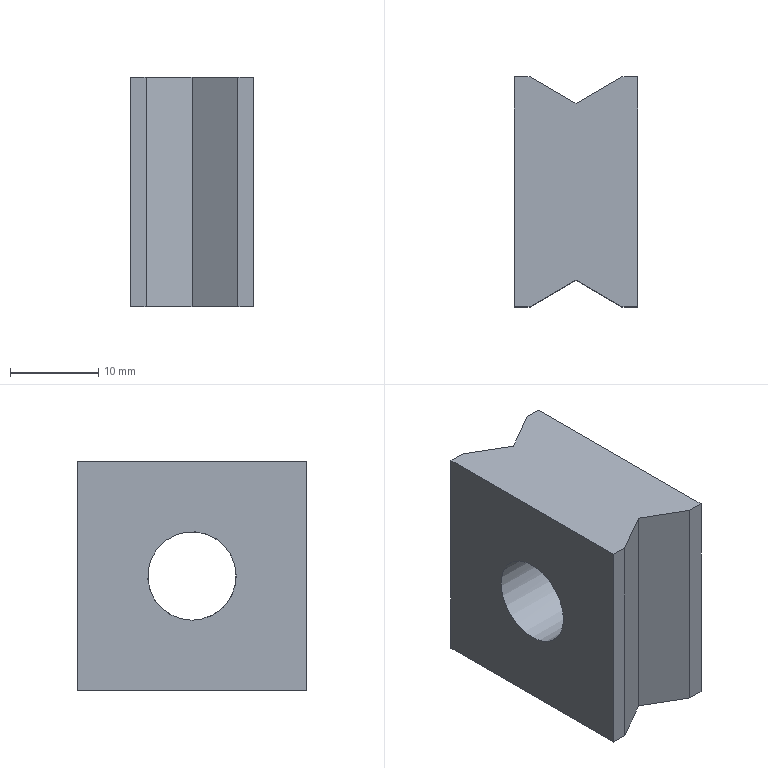Component | NX | 7_REVOLVING_LIFT_SLIDER | 1 solid | 13 faces | box 14 x 26 x 26 mm | volume 7554 mm3 | plane 12 | cylinder 1 | commonest cylinder face diameters 10 x1
STEP:
#1=CARTESIAN_POINT('',(0.,0.,0.));
#2=DIRECTION('',(0.,0.,1.));
#3=DIRECTION('',(1.,0.,0.));
#4=AXIS2_PLACEMENT_3D('',#1,#2,#3);
#5=CARTESIAN_POINT('',(29.804,13.,62.));
#6=VERTEX_POINT('',#5);
#7=CARTESIAN_POINT('',(28.,13.,62.));
#8=VERTEX_POINT('',#7);
#9=CARTESIAN_POINT('',(29.804,13.,62.));
#10=DIRECTION('',(-1.,-0.,0.));
#11=VECTOR('',#10,1.);
#12=LINE('',#9,#11);
#13=CARTESIAN_POINT('',(29.804,13.,88.));
#14=DIRECTION('',(0.,-1.,0.));
#15=DIRECTION('',(1.,0.,0.));
#16=AXIS2_PLACEMENT_3D('',#13,#14,#15);
#17=PLANE('',#16);
#18=CARTESIAN_POINT('',(0.,-26.));
#19=DIRECTION('',(-1.,0.));
#20=VECTOR('',#19,1.);
#21=LINE('',#18,#20);
#22=(GEOMETRIC_REPRESENTATION_CONTEXT(2)PARAMETRIC_REPRESENTATION_CONTEXT()REPRESENTATION_CONTEXT('',''));
#23=DEFINITIONAL_REPRESENTATION('',(#21),#22);
#24=PCURVE('',#17,#23);
#25=CARTESIAN_POINT('',(35.,-0.,62.));
#26=DIRECTION('',(0.,0.,1.));
#27=DIRECTION('',(0.,-1.,0.));
#28=AXIS2_PLACEMENT_3D('',#25,#26,#27);
#29=PLANE('',#28);
#30=CARTESIAN_POINT('',(-13.,-5.196));
#31=DIRECTION('',(0.,-1.));
#32=VECTOR('',#31,1.);
#33=LINE('',#30,#32);
#34=(GEOMETRIC_REPRESENTATION_CONTEXT(2)PARAMETRIC_REPRESENTATION_CONTEXT()REPRESENTATION_CONTEXT('',''));
#35=DEFINITIONAL_REPRESENTATION('',(#33),#34);
#36=PCURVE('',#29,#35);
#37=SURFACE_CURVE('',#12,(#24,#36),.PCURVE_S1.);
#38=EDGE_CURVE('',#6,#8,#37,.T.);
#39=ORIENTED_EDGE('',*,*,#38,.T.);
#40=CARTESIAN_POINT('',(28.,13.,88.));
#41=VERTEX_POINT('',#40);
#42=CARTESIAN_POINT('',(28.,13.,88.));
#43=DIRECTION('',(0.,0.,-1.));
#44=VECTOR('',#43,1.);
#45=LINE('',#42,#44);
#46=CARTESIAN_POINT('',(-1.804,0.));
#47=DIRECTION('',(0.,-1.));
#48=VECTOR('',#47,1.);
#49=LINE('',#46,#48);
#50=(GEOMETRIC_REPRESENTATION_CONTEXT(2)PARAMETRIC_REPRESENTATION_CONTEXT()REPRESENTATION_CONTEXT('',''));
#51=DEFINITIONAL_REPRESENTATION('',(#49),#50);
#52=PCURVE('',#17,#51);
#53=CARTESIAN_POINT('',(28.,13.,88.));
#54=DIRECTION('',(1.,0.,0.));
#55=DIRECTION('',(0.,0.,1.));
#56=AXIS2_PLACEMENT_3D('',#53,#54,#55);
#57=PLANE('',#56);
#58=CARTESIAN_POINT('',(0.,0.));
#59=DIRECTION('',(-1.,0.));
#60=VECTOR('',#59,1.);
#61=LINE('',#58,#60);
#62=(GEOMETRIC_REPRESENTATION_CONTEXT(2)PARAMETRIC_REPRESENTATION_CONTEXT()REPRESENTATION_CONTEXT('',''));
#63=DEFINITIONAL_REPRESENTATION('',(#61),#62);
#64=PCURVE('',#57,#63);
#65=SURFACE_CURVE('',#45,(#52,#64),.PCURVE_S1.);
#66=EDGE_CURVE('',#41,#8,#65,.T.);
#67=ORIENTED_EDGE('',*,*,#66,.F.);
#68=CARTESIAN_POINT('',(29.804,13.,88.));
#69=VERTEX_POINT('',#68);
#70=CARTESIAN_POINT('',(29.804,13.,88.));
#71=DIRECTION('',(-1.,-0.,0.));
#72=VECTOR('',#71,1.);
#73=LINE('',#70,#72);
#74=CARTESIAN_POINT('',(0.,0.));
#75=DIRECTION('',(-1.,0.));
#76=VECTOR('',#75,1.);
#77=LINE('',#74,#76);
#78=(GEOMETRIC_REPRESENTATION_CONTEXT(2)PARAMETRIC_REPRESENTATION_CONTEXT()REPRESENTATION_CONTEXT('',''));
#79=DEFINITIONAL_REPRESENTATION('',(#77),#78);
#80=PCURVE('',#17,#79);
#81=CARTESIAN_POINT('',(35.,-0.,88.));
#82=DIRECTION('',(0.,0.,1.));
#83=DIRECTION('',(0.,-1.,0.));
#84=AXIS2_PLACEMENT_3D('',#81,#82,#83);
#85=PLANE('',#84);
#86=CARTESIAN_POINT('',(-13.,-5.196));
#87=DIRECTION('',(0.,-1.));
#88=VECTOR('',#87,1.);
#89=LINE('',#86,#88);
#90=(GEOMETRIC_REPRESENTATION_CONTEXT(2)PARAMETRIC_REPRESENTATION_CONTEXT()REPRESENTATION_CONTEXT('',''));
#91=DEFINITIONAL_REPRESENTATION('',(#89),#90);
#92=PCURVE('',#85,#91);
#93=SURFACE_CURVE('',#73,(#80,#92),.PCURVE_S1.);
#94=EDGE_CURVE('',#69,#41,#93,.T.);
#95=ORIENTED_EDGE('',*,*,#94,.F.);
#96=CARTESIAN_POINT('',(29.804,13.,88.));
#97=DIRECTION('',(0.,0.,-1.));
#98=VECTOR('',#97,1.);
#99=LINE('',#96,#98);
#100=CARTESIAN_POINT('',(0.,0.));
#101=DIRECTION('',(0.,-1.));
#102=VECTOR('',#101,1.);
#103=LINE('',#100,#102);
#104=(GEOMETRIC_REPRESENTATION_CONTEXT(2)PARAMETRIC_REPRESENTATION_CONTEXT()REPRESENTATION_CONTEXT('',''));
#105=DEFINITIONAL_REPRESENTATION('',(#103),#104);
#106=PCURVE('',#17,#105);
#107=CARTESIAN_POINT('',(35.,10.,88.));
#108=DIRECTION('',(-0.5,-0.866,0.));
#109=DIRECTION('',(0.866,-0.5,0.));
#110=AXIS2_PLACEMENT_3D('',#107,#108,#109);
#111=PLANE('',#110);
#112=CARTESIAN_POINT('',(-6.,0.));
#113=DIRECTION('',(0.,-1.));
#114=VECTOR('',#113,1.);
#115=LINE('',#112,#114);
#116=(GEOMETRIC_REPRESENTATION_CONTEXT(2)PARAMETRIC_REPRESENTATION_CONTEXT()REPRESENTATION_CONTEXT('',''));
#117=DEFINITIONAL_REPRESENTATION('',(#115),#116);
#118=PCURVE('',#111,#117);
#119=SURFACE_CURVE('',#99,(#106,#118),.PCURVE_S1.);
#120=EDGE_CURVE('',#69,#6,#119,.T.);
#121=ORIENTED_EDGE('',*,*,#120,.T.);
#122=EDGE_LOOP('',(#39,#67,#95,#121));
#123=FACE_BOUND('',#122,.T.);
#124=ADVANCED_FACE('',(#123),#17,.F.);
#125=CARTESIAN_POINT('',(28.,-5.,75.));
#126=VERTEX_POINT('',#125);
#127=CARTESIAN_POINT('',(28.,-0.,70.));
#128=VERTEX_POINT('',#127);
#129=CARTESIAN_POINT('',(28.,-0.,75.));
#130=DIRECTION('',(-1.,0.,0.));
#131=DIRECTION('',(0.,-1.,0.));
#132=AXIS2_PLACEMENT_3D('',#129,#130,#131);
#133=CIRCLE('',#132,5.);
#134=CARTESIAN_POINT('',(-13.,18.));
#135=CARTESIAN_POINT('',(-4.34,18.));
#136=CARTESIAN_POINT('',(-8.67,10.5));
#137=CARTESIAN_POINT('',(-13.,3.));
#138=CARTESIAN_POINT('',(-17.33,10.5));
#139=CARTESIAN_POINT('',(-21.66,18.));
#140=CARTESIAN_POINT('',(-13.,18.));
#141=(BOUNDED_CURVE()B_SPLINE_CURVE(2,(#134,#135,#136,#137,#138,#139,#140),.UNSPECIFIED.,.T.,.F.)B_SPLINE_CURVE_WITH_KNOTS((1,2,2,2,2,1),(-2.094,0.,2.094,4.189,6.283,8.378),.UNSPECIFIED.)CURVE()GEOMETRIC_REPRESENTATION_ITEM()RATIONAL_B_SPLINE_CURVE((1.,0.5,1.,0.5,1.,0.5,1.))REPRESENTATION_ITEM(''));
#142=(GEOMETRIC_REPRESENTATION_CONTEXT(2)PARAMETRIC_REPRESENTATION_CONTEXT()REPRESENTATION_CONTEXT('',''));
#143=DEFINITIONAL_REPRESENTATION('',(#141),#142);
#144=PCURVE('',#57,#143);
#145=CARTESIAN_POINT('',(61.,-0.,75.));
#146=DIRECTION('',(-1.,0.,0.));
#147=DIRECTION('',(0.,0.,-1.));
#148=AXIS2_PLACEMENT_3D('',#145,#146,#147);
#149=CYLINDRICAL_SURFACE('',#148,5.);
#150=CARTESIAN_POINT('',(1.571,33.));
#151=DIRECTION('',(1.,0.));
#152=VECTOR('',#151,1.);
#153=LINE('',#150,#152);
#154=(GEOMETRIC_REPRESENTATION_CONTEXT(2)PARAMETRIC_REPRESENTATION_CONTEXT()REPRESENTATION_CONTEXT('',''));
#155=DEFINITIONAL_REPRESENTATION('',(#153),#154);
#156=PCURVE('',#149,#155);
#157=SURFACE_CURVE('',#133,(#144,#156),.PCURVE_S1.);
#158=EDGE_CURVE('',#126,#128,#157,.T.);
#159=ORIENTED_EDGE('',*,*,#158,.F.);
#160=CARTESIAN_POINT('',(28.,-0.,75.));
#161=DIRECTION('',(-1.,0.,0.));
#162=DIRECTION('',(0.,-1.,0.));
#163=AXIS2_PLACEMENT_3D('',#160,#161,#162);
#164=CIRCLE('',#163,5.);
#165=CARTESIAN_POINT('',(-13.,18.));
#166=CARTESIAN_POINT('',(-4.34,18.));
#167=CARTESIAN_POINT('',(-8.67,10.5));
#168=CARTESIAN_POINT('',(-13.,3.));
#169=CARTESIAN_POINT('',(-17.33,10.5));
#170=CARTESIAN_POINT('',(-21.66,18.));
#171=CARTESIAN_POINT('',(-13.,18.));
#172=(BOUNDED_CURVE()B_SPLINE_CURVE(2,(#165,#166,#167,#168,#169,#170,#171),.UNSPECIFIED.,.T.,.F.)B_SPLINE_CURVE_WITH_KNOTS((1,2,2,2,2,1),(-2.094,0.,2.094,4.189,6.283,8.378),.UNSPECIFIED.)CURVE()GEOMETRIC_REPRESENTATION_ITEM()RATIONAL_B_SPLINE_CURVE((1.,0.5,1.,0.5,1.,0.5,1.))REPRESENTATION_ITEM(''));
#173=(GEOMETRIC_REPRESENTATION_CONTEXT(2)PARAMETRIC_REPRESENTATION_CONTEXT()REPRESENTATION_CONTEXT('',''));
#174=DEFINITIONAL_REPRESENTATION('',(#172),#173);
#175=PCURVE('',#57,#174);
#176=CARTESIAN_POINT('',(-4.712,33.));
#177=DIRECTION('',(1.,0.));
#178=VECTOR('',#177,1.);
#179=LINE('',#176,#178);
#180=(GEOMETRIC_REPRESENTATION_CONTEXT(2)PARAMETRIC_REPRESENTATION_CONTEXT()REPRESENTATION_CONTEXT('',''));
#181=DEFINITIONAL_REPRESENTATION('',(#179),#180);
#182=PCURVE('',#149,#181);
#183=SURFACE_CURVE('',#164,(#175,#182),.PCURVE_S1.);
#184=EDGE_CURVE('',#128,#126,#183,.T.);
#185=ORIENTED_EDGE('',*,*,#184,.F.);
#186=EDGE_LOOP('',(#159,#185));
#187=FACE_BOUND('',#186,.T.);
#188=CARTESIAN_POINT('',(28.,-13.,62.));
#189=VERTEX_POINT('',#188);
#190=CARTESIAN_POINT('',(28.,13.,62.));
#191=DIRECTION('',(0.,-1.,0.));
#192=VECTOR('',#191,1.);
#193=LINE('',#190,#192);
#194=CARTESIAN_POINT('',(-26.,0.));
#195=DIRECTION('',(0.,1.));
#196=VECTOR('',#195,1.);
#197=LINE('',#194,#196);
#198=(GEOMETRIC_REPRESENTATION_CONTEXT(2)PARAMETRIC_REPRESENTATION_CONTEXT()REPRESENTATION_CONTEXT('',''));
#199=DEFINITIONAL_REPRESENTATION('',(#197),#198);
#200=PCURVE('',#57,#199);
#201=CARTESIAN_POINT('',(-13.,-7.));
#202=DIRECTION('',(1.,0.));
#203=VECTOR('',#202,1.);
#204=LINE('',#201,#203);
#205=(GEOMETRIC_REPRESENTATION_CONTEXT(2)PARAMETRIC_REPRESENTATION_CONTEXT()REPRESENTATION_CONTEXT('',''));
#206=DEFINITIONAL_REPRESENTATION('',(#204),#205);
#207=PCURVE('',#29,#206);
#208=SURFACE_CURVE('',#193,(#200,#207),.PCURVE_S1.);
#209=EDGE_CURVE('',#8,#189,#208,.T.);
#210=ORIENTED_EDGE('',*,*,#209,.T.);
#211=CARTESIAN_POINT('',(28.,-13.,88.));
#212=VERTEX_POINT('',#211);
#213=CARTESIAN_POINT('',(28.,-13.,88.));
#214=DIRECTION('',(0.,0.,-1.));
#215=VECTOR('',#214,1.);
#216=LINE('',#213,#215);
#217=CARTESIAN_POINT('',(0.,26.));
#218=DIRECTION('',(-1.,0.));
#219=VECTOR('',#218,1.);
#220=LINE('',#217,#219);
#221=(GEOMETRIC_REPRESENTATION_CONTEXT(2)PARAMETRIC_REPRESENTATION_CONTEXT()REPRESENTATION_CONTEXT('',''));
#222=DEFINITIONAL_REPRESENTATION('',(#220),#221);
#223=PCURVE('',#57,#222);
#224=CARTESIAN_POINT('',(28.,-13.,88.));
#225=DIRECTION('',(0.,1.,0.));
#226=DIRECTION('',(0.,0.,1.));
#227=AXIS2_PLACEMENT_3D('',#224,#225,#226);
#228=PLANE('',#227);
#229=CARTESIAN_POINT('',(0.,0.));
#230=DIRECTION('',(-1.,0.));
#231=VECTOR('',#230,1.);
#232=LINE('',#229,#231);
#233=(GEOMETRIC_REPRESENTATION_CONTEXT(2)PARAMETRIC_REPRESENTATION_CONTEXT()REPRESENTATION_CONTEXT('',''));
#234=DEFINITIONAL_REPRESENTATION('',(#232),#233);
#235=PCURVE('',#228,#234);
#236=SURFACE_CURVE('',#216,(#223,#235),.PCURVE_S1.);
#237=EDGE_CURVE('',#212,#189,#236,.T.);
#238=ORIENTED_EDGE('',*,*,#237,.F.);
#239=CARTESIAN_POINT('',(28.,13.,88.));
#240=DIRECTION('',(0.,-1.,0.));
#241=VECTOR('',#240,1.);
#242=LINE('',#239,#241);
#243=CARTESIAN_POINT('',(0.,0.));
#244=DIRECTION('',(0.,1.));
#245=VECTOR('',#244,1.);
#246=LINE('',#243,#245);
#247=(GEOMETRIC_REPRESENTATION_CONTEXT(2)PARAMETRIC_REPRESENTATION_CONTEXT()REPRESENTATION_CONTEXT('',''));
#248=DEFINITIONAL_REPRESENTATION('',(#246),#247);
#249=PCURVE('',#57,#248);
#250=CARTESIAN_POINT('',(-13.,-7.));
#251=DIRECTION('',(1.,0.));
#252=VECTOR('',#251,1.);
#253=LINE('',#250,#252);
#254=(GEOMETRIC_REPRESENTATION_CONTEXT(2)PARAMETRIC_REPRESENTATION_CONTEXT()REPRESENTATION_CONTEXT('',''));
#255=DEFINITIONAL_REPRESENTATION('',(#253),#254);
#256=PCURVE('',#85,#255);
#257=SURFACE_CURVE('',#242,(#249,#256),.PCURVE_S1.);
#258=EDGE_CURVE('',#41,#212,#257,.T.);
#259=ORIENTED_EDGE('',*,*,#258,.F.);
#260=ORIENTED_EDGE('',*,*,#66,.T.);
#261=EDGE_LOOP('',(#210,#238,#259,#260));
#262=FACE_BOUND('',#261,.T.);
#263=ADVANCED_FACE('',(#187,#262),#57,.F.);
#264=CARTESIAN_POINT('',(29.804,-13.,62.));
#265=VERTEX_POINT('',#264);
#266=CARTESIAN_POINT('',(28.,-13.,62.));
#267=DIRECTION('',(1.,0.,0.));
#268=VECTOR('',#267,1.);
#269=LINE('',#266,#268);
#270=CARTESIAN_POINT('',(-26.,0.));
#271=DIRECTION('',(0.,1.));
#272=VECTOR('',#271,1.);
#273=LINE('',#270,#272);
#274=(GEOMETRIC_REPRESENTATION_CONTEXT(2)PARAMETRIC_REPRESENTATION_CONTEXT()REPRESENTATION_CONTEXT('',''));
#275=DEFINITIONAL_REPRESENTATION('',(#273),#274);
#276=PCURVE('',#228,#275);
#277=CARTESIAN_POINT('',(13.,-7.));
#278=DIRECTION('',(0.,1.));
#279=VECTOR('',#278,1.);
#280=LINE('',#277,#279);
#281=(GEOMETRIC_REPRESENTATION_CONTEXT(2)PARAMETRIC_REPRESENTATION_CONTEXT()REPRESENTATION_CONTEXT('',''));
#282=DEFINITIONAL_REPRESENTATION('',(#280),#281);
#283=PCURVE('',#29,#282);
#284=SURFACE_CURVE('',#269,(#276,#283),.PCURVE_S1.);
#285=EDGE_CURVE('',#189,#265,#284,.T.);
#286=ORIENTED_EDGE('',*,*,#285,.T.);
#287=CARTESIAN_POINT('',(29.804,-13.,88.));
#288=VERTEX_POINT('',#287);
#289=CARTESIAN_POINT('',(29.804,-13.,88.));
#290=DIRECTION('',(0.,0.,-1.));
#291=VECTOR('',#290,1.);
#292=LINE('',#289,#291);
#293=CARTESIAN_POINT('',(0.,1.804));
#294=DIRECTION('',(-1.,0.));
#295=VECTOR('',#294,1.);
#296=LINE('',#293,#295);
#297=(GEOMETRIC_REPRESENTATION_CONTEXT(2)PARAMETRIC_REPRESENTATION_CONTEXT()REPRESENTATION_CONTEXT('',''));
#298=DEFINITIONAL_REPRESENTATION('',(#296),#297);
#299=PCURVE('',#228,#298);
#300=CARTESIAN_POINT('',(29.804,-13.,88.));
#301=DIRECTION('',(-0.5,0.866,0.));
#302=DIRECTION('',(-0.866,-0.5,0.));
#303=AXIS2_PLACEMENT_3D('',#300,#301,#302);
#304=PLANE('',#303);
#305=CARTESIAN_POINT('',(0.,0.));
#306=DIRECTION('',(0.,-1.));
#307=VECTOR('',#306,1.);
#308=LINE('',#305,#307);
#309=(GEOMETRIC_REPRESENTATION_CONTEXT(2)PARAMETRIC_REPRESENTATION_CONTEXT()REPRESENTATION_CONTEXT('',''));
#310=DEFINITIONAL_REPRESENTATION('',(#308),#309);
#311=PCURVE('',#304,#310);
#312=SURFACE_CURVE('',#292,(#299,#311),.PCURVE_S1.);
#313=EDGE_CURVE('',#288,#265,#312,.T.);
#314=ORIENTED_EDGE('',*,*,#313,.F.);
#315=CARTESIAN_POINT('',(28.,-13.,88.));
#316=DIRECTION('',(1.,0.,0.));
#317=VECTOR('',#316,1.);
#318=LINE('',#315,#317);
#319=CARTESIAN_POINT('',(0.,0.));
#320=DIRECTION('',(0.,1.));
#321=VECTOR('',#320,1.);
#322=LINE('',#319,#321);
#323=(GEOMETRIC_REPRESENTATION_CONTEXT(2)PARAMETRIC_REPRESENTATION_CONTEXT()REPRESENTATION_CONTEXT('',''));
#324=DEFINITIONAL_REPRESENTATION('',(#322),#323);
#325=PCURVE('',#228,#324);
#326=CARTESIAN_POINT('',(13.,-7.));
#327=DIRECTION('',(0.,1.));
#328=VECTOR('',#327,1.);
#329=LINE('',#326,#328);
#330=(GEOMETRIC_REPRESENTATION_CONTEXT(2)PARAMETRIC_REPRESENTATION_CONTEXT()REPRESENTATION_CONTEXT('',''));
#331=DEFINITIONAL_REPRESENTATION('',(#329),#330);
#332=PCURVE('',#85,#331);
#333=SURFACE_CURVE('',#318,(#325,#332),.PCURVE_S1.);
#334=EDGE_CURVE('',#212,#288,#333,.T.);
#335=ORIENTED_EDGE('',*,*,#334,.F.);
#336=ORIENTED_EDGE('',*,*,#237,.T.);
#337=EDGE_LOOP('',(#286,#314,#335,#336));
#338=FACE_BOUND('',#337,.T.);
#339=ADVANCED_FACE('',(#338),#228,.F.);
#340=CARTESIAN_POINT('',(35.,-10.,62.));
#341=VERTEX_POINT('',#340);
#342=CARTESIAN_POINT('',(29.804,-13.,62.));
#343=DIRECTION('',(0.866,0.5,0.));
#344=VECTOR('',#343,1.);
#345=LINE('',#342,#344);
#346=CARTESIAN_POINT('',(0.,-26.));
#347=DIRECTION('',(-1.,0.));
#348=VECTOR('',#347,1.);
#349=LINE('',#346,#348);
#350=(GEOMETRIC_REPRESENTATION_CONTEXT(2)PARAMETRIC_REPRESENTATION_CONTEXT()REPRESENTATION_CONTEXT('',''));
#351=DEFINITIONAL_REPRESENTATION('',(#349),#350);
#352=PCURVE('',#304,#351);
#353=CARTESIAN_POINT('',(13.,-5.196));
#354=DIRECTION('',(-0.5,0.866));
#355=VECTOR('',#354,1.);
#356=LINE('',#353,#355);
#357=(GEOMETRIC_REPRESENTATION_CONTEXT(2)PARAMETRIC_REPRESENTATION_CONTEXT()REPRESENTATION_CONTEXT('',''));
#358=DEFINITIONAL_REPRESENTATION('',(#356),#357);
#359=PCURVE('',#29,#358);
#360=SURFACE_CURVE('',#345,(#352,#359),.PCURVE_S1.);
#361=EDGE_CURVE('',#265,#341,#360,.T.);
#362=ORIENTED_EDGE('',*,*,#361,.T.);
#363=CARTESIAN_POINT('',(35.,-10.,88.));
#364=VERTEX_POINT('',#363);
#365=CARTESIAN_POINT('',(35.,-10.,88.));
#366=DIRECTION('',(0.,0.,-1.));
#367=VECTOR('',#366,1.);
#368=LINE('',#365,#367);
#369=CARTESIAN_POINT('',(-6.,0.));
#370=DIRECTION('',(0.,-1.));
#371=VECTOR('',#370,1.);
#372=LINE('',#369,#371);
#373=(GEOMETRIC_REPRESENTATION_CONTEXT(2)PARAMETRIC_REPRESENTATION_CONTEXT()REPRESENTATION_CONTEXT('',''));
#374=DEFINITIONAL_REPRESENTATION('',(#372),#373);
#375=PCURVE('',#304,#374);
#376=CARTESIAN_POINT('',(35.,-10.,88.));
#377=DIRECTION('',(0.5,0.866,0.));
#378=DIRECTION('',(-0.866,0.5,0.));
#379=AXIS2_PLACEMENT_3D('',#376,#377,#378);
#380=PLANE('',#379);
#381=CARTESIAN_POINT('',(0.,0.));
#382=DIRECTION('',(0.,-1.));
#383=VECTOR('',#382,1.);
#384=LINE('',#381,#383);
#385=(GEOMETRIC_REPRESENTATION_CONTEXT(2)PARAMETRIC_REPRESENTATION_CONTEXT()REPRESENTATION_CONTEXT('',''));
#386=DEFINITIONAL_REPRESENTATION('',(#384),#385);
#387=PCURVE('',#380,#386);
#388=SURFACE_CURVE('',#368,(#375,#387),.PCURVE_S1.);
#389=EDGE_CURVE('',#364,#341,#388,.T.);
#390=ORIENTED_EDGE('',*,*,#389,.F.);
#391=CARTESIAN_POINT('',(29.804,-13.,88.));
#392=DIRECTION('',(0.866,0.5,0.));
#393=VECTOR('',#392,1.);
#394=LINE('',#391,#393);
#395=CARTESIAN_POINT('',(0.,0.));
#396=DIRECTION('',(-1.,0.));
#397=VECTOR('',#396,1.);
#398=LINE('',#395,#397);
#399=(GEOMETRIC_REPRESENTATION_CONTEXT(2)PARAMETRIC_REPRESENTATION_CONTEXT()REPRESENTATION_CONTEXT('',''));
#400=DEFINITIONAL_REPRESENTATION('',(#398),#399);
#401=PCURVE('',#304,#400);
#402=CARTESIAN_POINT('',(13.,-5.196));
#403=DIRECTION('',(-0.5,0.866));
#404=VECTOR('',#403,1.);
#405=LINE('',#402,#404);
#406=(GEOMETRIC_REPRESENTATION_CONTEXT(2)PARAMETRIC_REPRESENTATION_CONTEXT()REPRESENTATION_CONTEXT('',''));
#407=DEFINITIONAL_REPRESENTATION('',(#405),#406);
#408=PCURVE('',#85,#407);
#409=SURFACE_CURVE('',#394,(#401,#408),.PCURVE_S1.);
#410=EDGE_CURVE('',#288,#364,#409,.T.);
#411=ORIENTED_EDGE('',*,*,#410,.F.);
#412=ORIENTED_EDGE('',*,*,#313,.T.);
#413=EDGE_LOOP('',(#362,#390,#411,#412));
#414=FACE_BOUND('',#413,.T.);
#415=ADVANCED_FACE('',(#414),#304,.F.);
#416=CARTESIAN_POINT('',(40.196,-13.,62.));
#417=VERTEX_POINT('',#416);
#418=CARTESIAN_POINT('',(35.,-10.,62.));
#419=DIRECTION('',(0.866,-0.5,0.));
#420=VECTOR('',#419,1.);
#421=LINE('',#418,#420);
#422=CARTESIAN_POINT('',(0.,-26.));
#423=DIRECTION('',(-1.,0.));
#424=VECTOR('',#423,1.);
#425=LINE('',#422,#424);
#426=(GEOMETRIC_REPRESENTATION_CONTEXT(2)PARAMETRIC_REPRESENTATION_CONTEXT()REPRESENTATION_CONTEXT('',''));
#427=DEFINITIONAL_REPRESENTATION('',(#425),#426);
#428=PCURVE('',#380,#427);
#429=CARTESIAN_POINT('',(10.,0.));
#430=DIRECTION('',(0.5,0.866));
#431=VECTOR('',#430,1.);
#432=LINE('',#429,#431);
#433=(GEOMETRIC_REPRESENTATION_CONTEXT(2)PARAMETRIC_REPRESENTATION_CONTEXT()REPRESENTATION_CONTEXT('',''));
#434=DEFINITIONAL_REPRESENTATION('',(#432),#433);
#435=PCURVE('',#29,#434);
#436=SURFACE_CURVE('',#421,(#428,#435),.PCURVE_S1.);
#437=EDGE_CURVE('',#341,#417,#436,.T.);
#438=ORIENTED_EDGE('',*,*,#437,.T.);
#439=CARTESIAN_POINT('',(40.196,-13.,88.));
#440=VERTEX_POINT('',#439);
#441=CARTESIAN_POINT('',(40.196,-13.,88.));
#442=DIRECTION('',(0.,0.,-1.));
#443=VECTOR('',#442,1.);
#444=LINE('',#441,#443);
#445=CARTESIAN_POINT('',(-6.,0.));
#446=DIRECTION('',(0.,-1.));
#447=VECTOR('',#446,1.);
#448=LINE('',#445,#447);
#449=(GEOMETRIC_REPRESENTATION_CONTEXT(2)PARAMETRIC_REPRESENTATION_CONTEXT()REPRESENTATION_CONTEXT('',''));
#450=DEFINITIONAL_REPRESENTATION('',(#448),#449);
#451=PCURVE('',#380,#450);
#452=CARTESIAN_POINT('',(40.196,-13.,88.));
#453=DIRECTION('',(0.,1.,0.));
#454=DIRECTION('',(0.,0.,1.));
#455=AXIS2_PLACEMENT_3D('',#452,#453,#454);
#456=PLANE('',#455);
#457=CARTESIAN_POINT('',(0.,0.));
#458=DIRECTION('',(-1.,0.));
#459=VECTOR('',#458,1.);
#460=LINE('',#457,#459);
#461=(GEOMETRIC_REPRESENTATION_CONTEXT(2)PARAMETRIC_REPRESENTATION_CONTEXT()REPRESENTATION_CONTEXT('',''));
#462=DEFINITIONAL_REPRESENTATION('',(#460),#461);
#463=PCURVE('',#456,#462);
#464=SURFACE_CURVE('',#444,(#451,#463),.PCURVE_S1.);
#465=EDGE_CURVE('',#440,#417,#464,.T.);
#466=ORIENTED_EDGE('',*,*,#465,.F.);
#467=CARTESIAN_POINT('',(35.,-10.,88.));
#468=DIRECTION('',(0.866,-0.5,0.));
#469=VECTOR('',#468,1.);
#470=LINE('',#467,#469);
#471=CARTESIAN_POINT('',(0.,0.));
#472=DIRECTION('',(-1.,0.));
#473=VECTOR('',#472,1.);
#474=LINE('',#471,#473);
#475=(GEOMETRIC_REPRESENTATION_CONTEXT(2)PARAMETRIC_REPRESENTATION_CONTEXT()REPRESENTATION_CONTEXT('',''));
#476=DEFINITIONAL_REPRESENTATION('',(#474),#475);
#477=PCURVE('',#380,#476);
#478=CARTESIAN_POINT('',(10.,0.));
#479=DIRECTION('',(0.5,0.866));
#480=VECTOR('',#479,1.);
#481=LINE('',#478,#480);
#482=(GEOMETRIC_REPRESENTATION_CONTEXT(2)PARAMETRIC_REPRESENTATION_CONTEXT()REPRESENTATION_CONTEXT('',''));
#483=DEFINITIONAL_REPRESENTATION('',(#481),#482);
#484=PCURVE('',#85,#483);
#485=SURFACE_CURVE('',#470,(#477,#484),.PCURVE_S1.);
#486=EDGE_CURVE('',#364,#440,#485,.T.);
#487=ORIENTED_EDGE('',*,*,#486,.F.);
#488=ORIENTED_EDGE('',*,*,#389,.T.);
#489=EDGE_LOOP('',(#438,#466,#487,#488));
#490=FACE_BOUND('',#489,.T.);
#491=ADVANCED_FACE('',(#490),#380,.F.);
#492=CARTESIAN_POINT('',(42.,-13.,62.));
#493=VERTEX_POINT('',#492);
#494=CARTESIAN_POINT('',(40.196,-13.,62.));
#495=DIRECTION('',(1.,0.,0.));
#496=VECTOR('',#495,1.);
#497=LINE('',#494,#496);
#498=CARTESIAN_POINT('',(-26.,0.));
#499=DIRECTION('',(0.,1.));
#500=VECTOR('',#499,1.);
#501=LINE('',#498,#500);
#502=(GEOMETRIC_REPRESENTATION_CONTEXT(2)PARAMETRIC_REPRESENTATION_CONTEXT()REPRESENTATION_CONTEXT('',''));
#503=DEFINITIONAL_REPRESENTATION('',(#501),#502);
#504=PCURVE('',#456,#503);
#505=CARTESIAN_POINT('',(13.,5.196));
#506=DIRECTION('',(0.,1.));
#507=VECTOR('',#506,1.);
#508=LINE('',#505,#507);
#509=(GEOMETRIC_REPRESENTATION_CONTEXT(2)PARAMETRIC_REPRESENTATION_CONTEXT()REPRESENTATION_CONTEXT('',''));
#510=DEFINITIONAL_REPRESENTATION('',(#508),#509);
#511=PCURVE('',#29,#510);
#512=SURFACE_CURVE('',#497,(#504,#511),.PCURVE_S1.);
#513=EDGE_CURVE('',#417,#493,#512,.T.);
#514=ORIENTED_EDGE('',*,*,#513,.T.);
#515=CARTESIAN_POINT('',(42.,-13.,88.));
#516=VERTEX_POINT('',#515);
#517=CARTESIAN_POINT('',(42.,-13.,88.));
#518=DIRECTION('',(0.,0.,-1.));
#519=VECTOR('',#518,1.);
#520=LINE('',#517,#519);
#521=CARTESIAN_POINT('',(0.,1.804));
#522=DIRECTION('',(-1.,0.));
#523=VECTOR('',#522,1.);
#524=LINE('',#521,#523);
#525=(GEOMETRIC_REPRESENTATION_CONTEXT(2)PARAMETRIC_REPRESENTATION_CONTEXT()REPRESENTATION_CONTEXT('',''));
#526=DEFINITIONAL_REPRESENTATION('',(#524),#525);
#527=PCURVE('',#456,#526);
#528=CARTESIAN_POINT('',(42.,-13.,88.));
#529=DIRECTION('',(-1.,0.,0.));
#530=DIRECTION('',(0.,0.,-1.));
#531=AXIS2_PLACEMENT_3D('',#528,#529,#530);
#532=PLANE('',#531);
#533=CARTESIAN_POINT('',(0.,0.));
#534=DIRECTION('',(1.,0.));
#535=VECTOR('',#534,1.);
#536=LINE('',#533,#535);
#537=(GEOMETRIC_REPRESENTATION_CONTEXT(2)PARAMETRIC_REPRESENTATION_CONTEXT()REPRESENTATION_CONTEXT('',''));
#538=DEFINITIONAL_REPRESENTATION('',(#536),#537);
#539=PCURVE('',#532,#538);
#540=SURFACE_CURVE('',#520,(#527,#539),.PCURVE_S1.);
#541=EDGE_CURVE('',#516,#493,#540,.T.);
#542=ORIENTED_EDGE('',*,*,#541,.F.);
#543=CARTESIAN_POINT('',(40.196,-13.,88.));
#544=DIRECTION('',(1.,0.,0.));
#545=VECTOR('',#544,1.);
#546=LINE('',#543,#545);
#547=CARTESIAN_POINT('',(0.,0.));
#548=DIRECTION('',(0.,1.));
#549=VECTOR('',#548,1.);
#550=LINE('',#547,#549);
#551=(GEOMETRIC_REPRESENTATION_CONTEXT(2)PARAMETRIC_REPRESENTATION_CONTEXT()REPRESENTATION_CONTEXT('',''));
#552=DEFINITIONAL_REPRESENTATION('',(#550),#551);
#553=PCURVE('',#456,#552);
#554=CARTESIAN_POINT('',(13.,5.196));
#555=DIRECTION('',(0.,1.));
#556=VECTOR('',#555,1.);
#557=LINE('',#554,#556);
#558=(GEOMETRIC_REPRESENTATION_CONTEXT(2)PARAMETRIC_REPRESENTATION_CONTEXT()REPRESENTATION_CONTEXT('',''));
#559=DEFINITIONAL_REPRESENTATION('',(#557),#558);
#560=PCURVE('',#85,#559);
#561=SURFACE_CURVE('',#546,(#553,#560),.PCURVE_S1.);
#562=EDGE_CURVE('',#440,#516,#561,.T.);
#563=ORIENTED_EDGE('',*,*,#562,.F.);
#564=ORIENTED_EDGE('',*,*,#465,.T.);
#565=EDGE_LOOP('',(#514,#542,#563,#564));
#566=FACE_BOUND('',#565,.T.);
#567=ADVANCED_FACE('',(#566),#456,.F.);
#568=CARTESIAN_POINT('',(42.,-0.,70.));
#569=VERTEX_POINT('',#568);
#570=CARTESIAN_POINT('',(42.,-0.,75.));
#571=DIRECTION('',(-1.,0.,0.));
#572=DIRECTION('',(0.,0.,-1.));
#573=AXIS2_PLACEMENT_3D('',#570,#571,#572);
#574=CIRCLE('',#573,5.);
#575=CARTESIAN_POINT('',(13.,-13.));
#576=DIRECTION('',(1.,0.));
#577=AXIS2_PLACEMENT_2D('',#575,#576);
#578=CIRCLE('',#577,5.);
#579=(GEOMETRIC_REPRESENTATION_CONTEXT(2)PARAMETRIC_REPRESENTATION_CONTEXT()REPRESENTATION_CONTEXT('',''));
#580=DEFINITIONAL_REPRESENTATION('',(#578),#579);
#581=PCURVE('',#532,#580);
#582=CARTESIAN_POINT('',(0.,19.));
#583=DIRECTION('',(1.,0.));
#584=VECTOR('',#583,1.);
#585=LINE('',#582,#584);
#586=(GEOMETRIC_REPRESENTATION_CONTEXT(2)PARAMETRIC_REPRESENTATION_CONTEXT()REPRESENTATION_CONTEXT('',''));
#587=DEFINITIONAL_REPRESENTATION('',(#585),#586);
#588=PCURVE('',#149,#587);
#589=SURFACE_CURVE('',#574,(#581,#588),.PCURVE_S1.);
#590=EDGE_CURVE('',#569,#569,#589,.T.);
#591=ORIENTED_EDGE('',*,*,#590,.T.);
#592=EDGE_LOOP('',(#591));
#593=FACE_BOUND('',#592,.T.);
#594=CARTESIAN_POINT('',(42.,13.,62.));
#595=VERTEX_POINT('',#594);
#596=CARTESIAN_POINT('',(42.,-13.,62.));
#597=DIRECTION('',(0.,1.,0.));
#598=VECTOR('',#597,1.);
#599=LINE('',#596,#598);
#600=CARTESIAN_POINT('',(26.,0.));
#601=DIRECTION('',(0.,-1.));
#602=VECTOR('',#601,1.);
#603=LINE('',#600,#602);
#604=(GEOMETRIC_REPRESENTATION_CONTEXT(2)PARAMETRIC_REPRESENTATION_CONTEXT()REPRESENTATION_CONTEXT('',''));
#605=DEFINITIONAL_REPRESENTATION('',(#603),#604);
#606=PCURVE('',#532,#605);
#607=CARTESIAN_POINT('',(13.,7.));
#608=DIRECTION('',(-1.,0.));
#609=VECTOR('',#608,1.);
#610=LINE('',#607,#609);
#611=(GEOMETRIC_REPRESENTATION_CONTEXT(2)PARAMETRIC_REPRESENTATION_CONTEXT()REPRESENTATION_CONTEXT('',''));
#612=DEFINITIONAL_REPRESENTATION('',(#610),#611);
#613=PCURVE('',#29,#612);
#614=SURFACE_CURVE('',#599,(#606,#613),.PCURVE_S1.);
#615=EDGE_CURVE('',#493,#595,#614,.T.);
#616=ORIENTED_EDGE('',*,*,#615,.T.);
#617=CARTESIAN_POINT('',(42.,13.,88.));
#618=VERTEX_POINT('',#617);
#619=CARTESIAN_POINT('',(42.,13.,88.));
#620=DIRECTION('',(0.,0.,-1.));
#621=VECTOR('',#620,1.);
#622=LINE('',#619,#621);
#623=CARTESIAN_POINT('',(0.,-26.));
#624=DIRECTION('',(1.,0.));
#625=VECTOR('',#624,1.);
#626=LINE('',#623,#625);
#627=(GEOMETRIC_REPRESENTATION_CONTEXT(2)PARAMETRIC_REPRESENTATION_CONTEXT()REPRESENTATION_CONTEXT('',''));
#628=DEFINITIONAL_REPRESENTATION('',(#626),#627);
#629=PCURVE('',#532,#628);
#630=CARTESIAN_POINT('',(42.,13.,88.));
#631=DIRECTION('',(-0.,-1.,0.));
#632=DIRECTION('',(1.,-0.,0.));
#633=AXIS2_PLACEMENT_3D('',#630,#631,#632);
#634=PLANE('',#633);
#635=CARTESIAN_POINT('',(0.,0.));
#636=DIRECTION('',(0.,-1.));
#637=VECTOR('',#636,1.);
#638=LINE('',#635,#637);
#639=(GEOMETRIC_REPRESENTATION_CONTEXT(2)PARAMETRIC_REPRESENTATION_CONTEXT()REPRESENTATION_CONTEXT('',''));
#640=DEFINITIONAL_REPRESENTATION('',(#638),#639);
#641=PCURVE('',#634,#640);
#642=SURFACE_CURVE('',#622,(#629,#641),.PCURVE_S1.);
#643=EDGE_CURVE('',#618,#595,#642,.T.);
#644=ORIENTED_EDGE('',*,*,#643,.F.);
#645=CARTESIAN_POINT('',(42.,-13.,88.));
#646=DIRECTION('',(0.,1.,0.));
#647=VECTOR('',#646,1.);
#648=LINE('',#645,#647);
#649=CARTESIAN_POINT('',(0.,0.));
#650=DIRECTION('',(0.,-1.));
#651=VECTOR('',#650,1.);
#652=LINE('',#649,#651);
#653=(GEOMETRIC_REPRESENTATION_CONTEXT(2)PARAMETRIC_REPRESENTATION_CONTEXT()REPRESENTATION_CONTEXT('',''));
#654=DEFINITIONAL_REPRESENTATION('',(#652),#653);
#655=PCURVE('',#532,#654);
#656=CARTESIAN_POINT('',(13.,7.));
#657=DIRECTION('',(-1.,0.));
#658=VECTOR('',#657,1.);
#659=LINE('',#656,#658);
#660=(GEOMETRIC_REPRESENTATION_CONTEXT(2)PARAMETRIC_REPRESENTATION_CONTEXT()REPRESENTATION_CONTEXT('',''));
#661=DEFINITIONAL_REPRESENTATION('',(#659),#660);
#662=PCURVE('',#85,#661);
#663=SURFACE_CURVE('',#648,(#655,#662),.PCURVE_S1.);
#664=EDGE_CURVE('',#516,#618,#663,.T.);
#665=ORIENTED_EDGE('',*,*,#664,.F.);
#666=ORIENTED_EDGE('',*,*,#541,.T.);
#667=EDGE_LOOP('',(#616,#644,#665,#666));
#668=FACE_BOUND('',#667,.T.);
#669=ADVANCED_FACE('',(#593,#668),#532,.F.);
#670=CARTESIAN_POINT('',(40.196,13.,62.));
#671=VERTEX_POINT('',#670);
#672=CARTESIAN_POINT('',(42.,13.,62.));
#673=DIRECTION('',(-1.,0.,0.));
#674=VECTOR('',#673,1.);
#675=LINE('',#672,#674);
#676=CARTESIAN_POINT('',(0.,-26.));
#677=DIRECTION('',(-1.,0.));
#678=VECTOR('',#677,1.);
#679=LINE('',#676,#678);
#680=(GEOMETRIC_REPRESENTATION_CONTEXT(2)PARAMETRIC_REPRESENTATION_CONTEXT()REPRESENTATION_CONTEXT('',''));
#681=DEFINITIONAL_REPRESENTATION('',(#679),#680);
#682=PCURVE('',#634,#681);
#683=CARTESIAN_POINT('',(-13.,7.));
#684=DIRECTION('',(-0.,-1.));
#685=VECTOR('',#684,1.);
#686=LINE('',#683,#685);
#687=(GEOMETRIC_REPRESENTATION_CONTEXT(2)PARAMETRIC_REPRESENTATION_CONTEXT()REPRESENTATION_CONTEXT('',''));
#688=DEFINITIONAL_REPRESENTATION('',(#686),#687);
#689=PCURVE('',#29,#688);
#690=SURFACE_CURVE('',#675,(#682,#689),.PCURVE_S1.);
#691=EDGE_CURVE('',#595,#671,#690,.T.);
#692=ORIENTED_EDGE('',*,*,#691,.T.);
#693=CARTESIAN_POINT('',(40.196,13.,88.));
#694=VERTEX_POINT('',#693);
#695=CARTESIAN_POINT('',(40.196,13.,88.));
#696=DIRECTION('',(0.,0.,-1.));
#697=VECTOR('',#696,1.);
#698=LINE('',#695,#697);
#699=CARTESIAN_POINT('',(-1.804,0.));
#700=DIRECTION('',(0.,-1.));
#701=VECTOR('',#700,1.);
#702=LINE('',#699,#701);
#703=(GEOMETRIC_REPRESENTATION_CONTEXT(2)PARAMETRIC_REPRESENTATION_CONTEXT()REPRESENTATION_CONTEXT('',''));
#704=DEFINITIONAL_REPRESENTATION('',(#702),#703);
#705=PCURVE('',#634,#704);
#706=CARTESIAN_POINT('',(40.196,13.,88.));
#707=DIRECTION('',(0.5,-0.866,0.));
#708=DIRECTION('',(0.866,0.5,0.));
#709=AXIS2_PLACEMENT_3D('',#706,#707,#708);
#710=PLANE('',#709);
#711=CARTESIAN_POINT('',(0.,0.));
#712=DIRECTION('',(0.,-1.));
#713=VECTOR('',#712,1.);
#714=LINE('',#711,#713);
#715=(GEOMETRIC_REPRESENTATION_CONTEXT(2)PARAMETRIC_REPRESENTATION_CONTEXT()REPRESENTATION_CONTEXT('',''));
#716=DEFINITIONAL_REPRESENTATION('',(#714),#715);
#717=PCURVE('',#710,#716);
#718=SURFACE_CURVE('',#698,(#705,#717),.PCURVE_S1.);
#719=EDGE_CURVE('',#694,#671,#718,.T.);
#720=ORIENTED_EDGE('',*,*,#719,.F.);
#721=CARTESIAN_POINT('',(42.,13.,88.));
#722=DIRECTION('',(-1.,0.,0.));
#723=VECTOR('',#722,1.);
#724=LINE('',#721,#723);
#725=CARTESIAN_POINT('',(0.,0.));
#726=DIRECTION('',(-1.,0.));
#727=VECTOR('',#726,1.);
#728=LINE('',#725,#727);
#729=(GEOMETRIC_REPRESENTATION_CONTEXT(2)PARAMETRIC_REPRESENTATION_CONTEXT()REPRESENTATION_CONTEXT('',''));
#730=DEFINITIONAL_REPRESENTATION('',(#728),#729);
#731=PCURVE('',#634,#730);
#732=CARTESIAN_POINT('',(-13.,7.));
#733=DIRECTION('',(-0.,-1.));
#734=VECTOR('',#733,1.);
#735=LINE('',#732,#734);
#736=(GEOMETRIC_REPRESENTATION_CONTEXT(2)PARAMETRIC_REPRESENTATION_CONTEXT()REPRESENTATION_CONTEXT('',''));
#737=DEFINITIONAL_REPRESENTATION('',(#735),#736);
#738=PCURVE('',#85,#737);
#739=SURFACE_CURVE('',#724,(#731,#738),.PCURVE_S1.);
#740=EDGE_CURVE('',#618,#694,#739,.T.);
#741=ORIENTED_EDGE('',*,*,#740,.F.);
#742=ORIENTED_EDGE('',*,*,#643,.T.);
#743=EDGE_LOOP('',(#692,#720,#741,#742));
#744=FACE_BOUND('',#743,.T.);
#745=ADVANCED_FACE('',(#744),#634,.F.);
#746=CARTESIAN_POINT('',(35.,10.,62.));
#747=VERTEX_POINT('',#746);
#748=CARTESIAN_POINT('',(40.196,13.,62.));
#749=DIRECTION('',(-0.866,-0.5,0.));
#750=VECTOR('',#749,1.);
#751=LINE('',#748,#750);
#752=CARTESIAN_POINT('',(0.,-26.));
#753=DIRECTION('',(-1.,0.));
#754=VECTOR('',#753,1.);
#755=LINE('',#752,#754);
#756=(GEOMETRIC_REPRESENTATION_CONTEXT(2)PARAMETRIC_REPRESENTATION_CONTEXT()REPRESENTATION_CONTEXT('',''));
#757=DEFINITIONAL_REPRESENTATION('',(#755),#756);
#758=PCURVE('',#710,#757);
#759=CARTESIAN_POINT('',(-13.,5.196));
#760=DIRECTION('',(0.5,-0.866));
#761=VECTOR('',#760,1.);
#762=LINE('',#759,#761);
#763=(GEOMETRIC_REPRESENTATION_CONTEXT(2)PARAMETRIC_REPRESENTATION_CONTEXT()REPRESENTATION_CONTEXT('',''));
#764=DEFINITIONAL_REPRESENTATION('',(#762),#763);
#765=PCURVE('',#29,#764);
#766=SURFACE_CURVE('',#751,(#758,#765),.PCURVE_S1.);
#767=EDGE_CURVE('',#671,#747,#766,.T.);
#768=ORIENTED_EDGE('',*,*,#767,.T.);
#769=CARTESIAN_POINT('',(35.,10.,88.));
#770=VERTEX_POINT('',#769);
#771=CARTESIAN_POINT('',(35.,10.,88.));
#772=DIRECTION('',(0.,0.,-1.));
#773=VECTOR('',#772,1.);
#774=LINE('',#771,#773);
#775=CARTESIAN_POINT('',(-6.,0.));
#776=DIRECTION('',(0.,-1.));
#777=VECTOR('',#776,1.);
#778=LINE('',#775,#777);
#779=(GEOMETRIC_REPRESENTATION_CONTEXT(2)PARAMETRIC_REPRESENTATION_CONTEXT()REPRESENTATION_CONTEXT('',''));
#780=DEFINITIONAL_REPRESENTATION('',(#778),#779);
#781=PCURVE('',#710,#780);
#782=CARTESIAN_POINT('',(0.,0.));
#783=DIRECTION('',(0.,-1.));
#784=VECTOR('',#783,1.);
#785=LINE('',#782,#784);
#786=(GEOMETRIC_REPRESENTATION_CONTEXT(2)PARAMETRIC_REPRESENTATION_CONTEXT()REPRESENTATION_CONTEXT('',''));
#787=DEFINITIONAL_REPRESENTATION('',(#785),#786);
#788=PCURVE('',#111,#787);
#789=SURFACE_CURVE('',#774,(#781,#788),.PCURVE_S1.);
#790=EDGE_CURVE('',#770,#747,#789,.T.);
#791=ORIENTED_EDGE('',*,*,#790,.F.);
#792=CARTESIAN_POINT('',(40.196,13.,88.));
#793=DIRECTION('',(-0.866,-0.5,0.));
#794=VECTOR('',#793,1.);
#795=LINE('',#792,#794);
#796=CARTESIAN_POINT('',(0.,0.));
#797=DIRECTION('',(-1.,0.));
#798=VECTOR('',#797,1.);
#799=LINE('',#796,#798);
#800=(GEOMETRIC_REPRESENTATION_CONTEXT(2)PARAMETRIC_REPRESENTATION_CONTEXT()REPRESENTATION_CONTEXT('',''));
#801=DEFINITIONAL_REPRESENTATION('',(#799),#800);
#802=PCURVE('',#710,#801);
#803=CARTESIAN_POINT('',(-13.,5.196));
#804=DIRECTION('',(0.5,-0.866));
#805=VECTOR('',#804,1.);
#806=LINE('',#803,#805);
#807=(GEOMETRIC_REPRESENTATION_CONTEXT(2)PARAMETRIC_REPRESENTATION_CONTEXT()REPRESENTATION_CONTEXT('',''));
#808=DEFINITIONAL_REPRESENTATION('',(#806),#807);
#809=PCURVE('',#85,#808);
#810=SURFACE_CURVE('',#795,(#802,#809),.PCURVE_S1.);
#811=EDGE_CURVE('',#694,#770,#810,.T.);
#812=ORIENTED_EDGE('',*,*,#811,.F.);
#813=ORIENTED_EDGE('',*,*,#719,.T.);
#814=EDGE_LOOP('',(#768,#791,#812,#813));
#815=FACE_BOUND('',#814,.T.);
#816=ADVANCED_FACE('',(#815),#710,.F.);
#817=CARTESIAN_POINT('',(35.,10.,62.));
#818=DIRECTION('',(-0.866,0.5,0.));
#819=VECTOR('',#818,1.);
#820=LINE('',#817,#819);
#821=CARTESIAN_POINT('',(0.,-26.));
#822=DIRECTION('',(-1.,0.));
#823=VECTOR('',#822,1.);
#824=LINE('',#821,#823);
#825=(GEOMETRIC_REPRESENTATION_CONTEXT(2)PARAMETRIC_REPRESENTATION_CONTEXT()REPRESENTATION_CONTEXT('',''));
#826=DEFINITIONAL_REPRESENTATION('',(#824),#825);
#827=PCURVE('',#111,#826);
#828=CARTESIAN_POINT('',(-10.,0.));
#829=DIRECTION('',(-0.5,-0.866));
#830=VECTOR('',#829,1.);
#831=LINE('',#828,#830);
#832=(GEOMETRIC_REPRESENTATION_CONTEXT(2)PARAMETRIC_REPRESENTATION_CONTEXT()REPRESENTATION_CONTEXT('',''));
#833=DEFINITIONAL_REPRESENTATION('',(#831),#832);
#834=PCURVE('',#29,#833);
#835=SURFACE_CURVE('',#820,(#827,#834),.PCURVE_S1.);
#836=EDGE_CURVE('',#747,#6,#835,.T.);
#837=ORIENTED_EDGE('',*,*,#836,.T.);
#838=ORIENTED_EDGE('',*,*,#120,.F.);
#839=CARTESIAN_POINT('',(35.,10.,88.));
#840=DIRECTION('',(-0.866,0.5,0.));
#841=VECTOR('',#840,1.);
#842=LINE('',#839,#841);
#843=CARTESIAN_POINT('',(0.,0.));
#844=DIRECTION('',(-1.,0.));
#845=VECTOR('',#844,1.);
#846=LINE('',#843,#845);
#847=(GEOMETRIC_REPRESENTATION_CONTEXT(2)PARAMETRIC_REPRESENTATION_CONTEXT()REPRESENTATION_CONTEXT('',''));
#848=DEFINITIONAL_REPRESENTATION('',(#846),#847);
#849=PCURVE('',#111,#848);
#850=CARTESIAN_POINT('',(-10.,0.));
#851=DIRECTION('',(-0.5,-0.866));
#852=VECTOR('',#851,1.);
#853=LINE('',#850,#852);
#854=(GEOMETRIC_REPRESENTATION_CONTEXT(2)PARAMETRIC_REPRESENTATION_CONTEXT()REPRESENTATION_CONTEXT('',''));
#855=DEFINITIONAL_REPRESENTATION('',(#853),#854);
#856=PCURVE('',#85,#855);
#857=SURFACE_CURVE('',#842,(#849,#856),.PCURVE_S1.);
#858=EDGE_CURVE('',#770,#69,#857,.T.);
#859=ORIENTED_EDGE('',*,*,#858,.F.);
#860=ORIENTED_EDGE('',*,*,#790,.T.);
#861=EDGE_LOOP('',(#837,#838,#859,#860));
#862=FACE_BOUND('',#861,.T.);
#863=ADVANCED_FACE('',(#862),#111,.F.);
#864=ORIENTED_EDGE('',*,*,#94,.T.);
#865=ORIENTED_EDGE('',*,*,#258,.T.);
#866=ORIENTED_EDGE('',*,*,#334,.T.);
#867=ORIENTED_EDGE('',*,*,#410,.T.);
#868=ORIENTED_EDGE('',*,*,#486,.T.);
#869=ORIENTED_EDGE('',*,*,#562,.T.);
#870=ORIENTED_EDGE('',*,*,#664,.T.);
#871=ORIENTED_EDGE('',*,*,#740,.T.);
#872=ORIENTED_EDGE('',*,*,#811,.T.);
#873=ORIENTED_EDGE('',*,*,#858,.T.);
#874=EDGE_LOOP('',(#864,#865,#866,#867,#868,#869,#870,#871,#872,#873));
#875=FACE_BOUND('',#874,.T.);
#876=ADVANCED_FACE('',(#875),#85,.T.);
#877=ORIENTED_EDGE('',*,*,#38,.F.);
#878=ORIENTED_EDGE('',*,*,#836,.F.);
#879=ORIENTED_EDGE('',*,*,#767,.F.);
#880=ORIENTED_EDGE('',*,*,#691,.F.);
#881=ORIENTED_EDGE('',*,*,#615,.F.);
#882=ORIENTED_EDGE('',*,*,#513,.F.);
#883=ORIENTED_EDGE('',*,*,#437,.F.);
#884=ORIENTED_EDGE('',*,*,#361,.F.);
#885=ORIENTED_EDGE('',*,*,#285,.F.);
#886=ORIENTED_EDGE('',*,*,#209,.F.);
#887=EDGE_LOOP('',(#877,#878,#879,#880,#881,#882,#883,#884,#885,#886));
#888=FACE_BOUND('',#887,.T.);
#889=ADVANCED_FACE('',(#888),#29,.F.);
#890=ORIENTED_EDGE('',*,*,#184,.F.);
#891=CARTESIAN_POINT('',(42.,-0.,70.));
#892=CARTESIAN_POINT('',(28.,-0.,70.));
#893=B_SPLINE_CURVE_WITH_KNOTS('',1,(#891,#892),.UNSPECIFIED.,.F.,.F.,(2,2),(19.,33.),.PIECEWISE_BEZIER_KNOTS.);
#894=CARTESIAN_POINT('',(0.,0.));
#895=DIRECTION('',(0.,1.));
#896=VECTOR('',#895,1.);
#897=LINE('',#894,#896);
#898=(GEOMETRIC_REPRESENTATION_CONTEXT(2)PARAMETRIC_REPRESENTATION_CONTEXT()REPRESENTATION_CONTEXT('',''));
#899=DEFINITIONAL_REPRESENTATION('',(#897),#898);
#900=PCURVE('',#149,#899);
#901=CARTESIAN_POINT('',(6.283,0.));
#902=DIRECTION('',(0.,1.));
#903=VECTOR('',#902,1.);
#904=LINE('',#901,#903);
#905=(GEOMETRIC_REPRESENTATION_CONTEXT(2)PARAMETRIC_REPRESENTATION_CONTEXT()REPRESENTATION_CONTEXT('',''));
#906=DEFINITIONAL_REPRESENTATION('',(#904),#905);
#907=PCURVE('',#149,#906);
#908=SEAM_CURVE('',#893,(#900,#907),.PCURVE_S1.);
#909=EDGE_CURVE('',#569,#128,#908,.T.);
#910=ORIENTED_EDGE('',*,*,#909,.F.);
#911=ORIENTED_EDGE('',*,*,#590,.T.);
#912=ORIENTED_EDGE('',*,*,#909,.T.);
#913=ORIENTED_EDGE('',*,*,#158,.F.);
#914=EDGE_LOOP('',(#890,#910,#911,#912,#913));
#915=FACE_BOUND('',#914,.F.);
#916=ADVANCED_FACE('',(#915),#149,.F.);
#917=CLOSED_SHELL('',(#124,#263,#339,#415,#491,#567,#669,#745,#816,#863,#876,#889,#916));
#918=MANIFOLD_SOLID_BREP('',#917);
#919=(LENGTH_UNIT()NAMED_UNIT(*)SI_UNIT(.MILLI.,.METRE.));
#920=UNCERTAINTY_MEASURE_WITH_UNIT(LENGTH_MEASURE(0.000001),#919,'','');
#921=(NAMED_UNIT(*)PLANE_ANGLE_UNIT()SI_UNIT($,.RADIAN.));
#922=(NAMED_UNIT(*)SI_UNIT($,.STERADIAN.)SOLID_ANGLE_UNIT());
#923=(GEOMETRIC_REPRESENTATION_CONTEXT(3)GLOBAL_UNCERTAINTY_ASSIGNED_CONTEXT((#920))GLOBAL_UNIT_ASSIGNED_CONTEXT((#919,#921,#922))REPRESENTATION_CONTEXT('',''));
#924=ADVANCED_BREP_SHAPE_REPRESENTATION('',(#4,#918),#923);